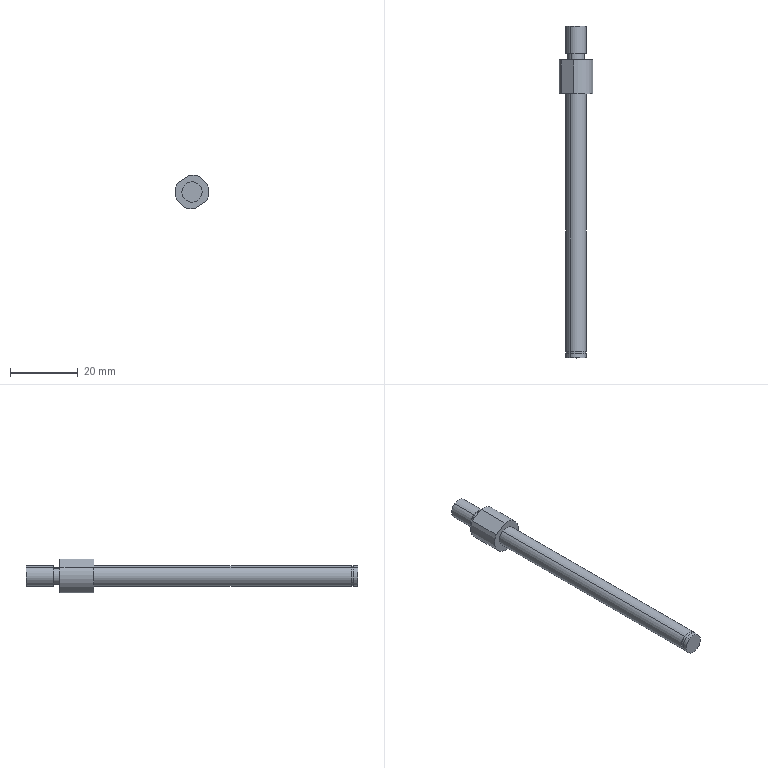Component | SolidWorks | JL001-03-06-1_JL001-03-06-001-1 | 1 solid | 21 faces | box 10 x 98 x 10 mm | volume 3225 mm3 | cylinder 12 | plane 9 | commonest cylinder face diameters 6 x6 5 x2 5.7 x2 10 x2
build123d program:
from build123d import *

# Parameters (mm, degrees)
SKETCH6_OUTSIDE_W   = 31.804
SKETCH6_OUTSIDE_H   = 31.804
SKETCH6_OUTSIDE_W_2 = 16.589
SKETCH6_OUTSIDE_H_2 = 9
CUT_EXTRUDE2_DEPTH  = 79.32


with BuildPart() as part:
    # Sketch1 → Revolve1 (revolve)
    with BuildSketch(Plane.XY, mode=Mode.PRIVATE) as revolve1_sk:
        Polygon((0, 98), (3, 98), (3, 96.8), (2.85, 96.8), (2.85, 96), (3, 96), (3, 20), (5, 20), (5, 10), (2.5, 10), (2.5, 8), (3, 8), (3, 0), (0, 0), align=None)
    revolve(revolve1_sk.sketch.rotate(Axis((0, 0, 0), (0, 1, 0)), 90), axis=Axis((0, 0, 0), (0, 1, 0)))

    # Sketch6 outside → Cut-Extrude2 (cut, through all)
    with BuildSketch(Plane(origin=(0, 20, 0), x_dir=(1, 0, 0), z_dir=(0, 1, 0))):
        Rectangle(SKETCH6_OUTSIDE_W, SKETCH6_OUTSIDE_H)
        Rectangle(SKETCH6_OUTSIDE_W_2, SKETCH6_OUTSIDE_H_2, mode=Mode.SUBTRACT)
    extrude(amount=-CUT_EXTRUDE2_DEPTH, mode=Mode.SUBTRACT)


solid = part.part

# Placed as in the assembly
solid = solid.moved(Location((-69, 1135, 65), (0, -33.158, 180)))
STEP:
#1=CARTESIAN_POINT('',(-2.781,44.37,2.658));
#2=VERTEX_POINT('',#1);
#3=CARTESIAN_POINT('',(-2.652,44.37,2.46));
#4=VERTEX_POINT('',#3);
#5=CARTESIAN_POINT('',(-2.717,44.37,2.559));
#6=DIRECTION('',(0.,1.,0.));
#7=DIRECTION('',(-0.5469,0.,0.8372));
#8=AXIS2_PLACEMENT_3D('',#5,#6,#7);
#9=CIRCLE('',#8,0.1181);
#10=EDGE_CURVE('',#2,#4,#9,.T.);
#11=ORIENTED_EDGE('',*,*,#10,.T.);
#12=CARTESIAN_POINT('',(-2.652,44.685,2.46));
#13=VERTEX_POINT('',#12);
#14=CARTESIAN_POINT('',(-2.652,44.685,2.46));
#15=DIRECTION('',(0.,1.,0.));
#16=VECTOR('',#15,39.37);
#17=LINE('',#14,#16);
#18=EDGE_CURVE('',#4,#13,#17,.T.);
#19=ORIENTED_EDGE('',*,*,#18,.T.);
#20=CARTESIAN_POINT('',(-2.781,44.685,2.658));
#21=VERTEX_POINT('',#20);
#22=CARTESIAN_POINT('',(-2.717,44.685,2.559));
#23=DIRECTION('',(0.,1.,0.));
#24=DIRECTION('',(-0.5469,0.,0.8372));
#25=AXIS2_PLACEMENT_3D('',#22,#23,#24);
#26=CIRCLE('',#25,0.1181);
#27=EDGE_CURVE('',#21,#13,#26,.T.);
#28=ORIENTED_EDGE('',*,*,#27,.F.);
#29=CARTESIAN_POINT('',(-2.781,44.685,2.658));
#30=DIRECTION('',(0.,1.,0.));
#31=VECTOR('',#30,39.37);
#32=LINE('',#29,#31);
#33=EDGE_CURVE('',#2,#21,#32,.T.);
#34=ORIENTED_EDGE('',*,*,#33,.F.);
#35=EDGE_LOOP('',(#11,#19,#28,#34));
#36=FACE_OUTER_BOUND('',#35,.T.);
#37=CARTESIAN_POINT('',(-2.717,44.685,2.559));
#38=DIRECTION('',(0.,1.,0.));
#39=DIRECTION('',(-0.5469,0.,0.8372));
#40=AXIS2_PLACEMENT_3D('',#37,#38,#39);
#41=CYLINDRICAL_SURFACE('',#40,0.1181);
#42=ADVANCED_FACE('',(#36),#41,.T.);
#43=CARTESIAN_POINT('',(-2.77,44.291,2.641));
#44=VERTEX_POINT('',#43);
#45=CARTESIAN_POINT('',(-2.663,44.291,2.477));
#46=VERTEX_POINT('',#45);
#47=CARTESIAN_POINT('',(-2.717,44.291,2.559));
#48=DIRECTION('',(0.,1.,0.));
#49=DIRECTION('',(-0.5469,0.,0.8372));
#50=AXIS2_PLACEMENT_3D('',#47,#48,#49);
#51=CIRCLE('',#50,0.09843);
#52=EDGE_CURVE('',#44,#46,#51,.T.);
#53=ORIENTED_EDGE('',*,*,#52,.T.);
#54=CARTESIAN_POINT('',(-2.663,44.37,2.477));
#55=VERTEX_POINT('',#54);
#56=CARTESIAN_POINT('',(-2.663,44.685,2.477));
#57=DIRECTION('',(0.,1.,0.));
#58=VECTOR('',#57,39.37);
#59=LINE('',#56,#58);
#60=EDGE_CURVE('',#46,#55,#59,.T.);
#61=ORIENTED_EDGE('',*,*,#60,.T.);
#62=CARTESIAN_POINT('',(-2.77,44.37,2.641));
#63=VERTEX_POINT('',#62);
#64=CARTESIAN_POINT('',(-2.717,44.37,2.559));
#65=DIRECTION('',(0.,1.,0.));
#66=DIRECTION('',(-0.5469,0.,0.8372));
#67=AXIS2_PLACEMENT_3D('',#64,#65,#66);
#68=CIRCLE('',#67,0.09843);
#69=EDGE_CURVE('',#63,#55,#68,.T.);
#70=ORIENTED_EDGE('',*,*,#69,.F.);
#71=CARTESIAN_POINT('',(-2.77,44.685,2.641));
#72=DIRECTION('',(0.,1.,0.));
#73=VECTOR('',#72,39.37);
#74=LINE('',#71,#73);
#75=EDGE_CURVE('',#44,#63,#74,.T.);
#76=ORIENTED_EDGE('',*,*,#75,.F.);
#77=EDGE_LOOP('',(#53,#61,#70,#76));
#78=FACE_OUTER_BOUND('',#77,.T.);
#79=CARTESIAN_POINT('',(-2.717,44.685,2.559));
#80=DIRECTION('',(0.,1.,0.));
#81=DIRECTION('',(-0.5469,0.,0.8372));
#82=AXIS2_PLACEMENT_3D('',#79,#80,#81);
#83=CYLINDRICAL_SURFACE('',#82,0.09843);
#84=ADVANCED_FACE('',(#78),#83,.T.);
#85=CARTESIAN_POINT('',(-2.781,40.906,2.658));
#86=VERTEX_POINT('',#85);
#87=CARTESIAN_POINT('',(-2.652,40.906,2.46));
#88=VERTEX_POINT('',#87);
#89=CARTESIAN_POINT('',(-2.717,40.906,2.559));
#90=DIRECTION('',(0.,1.,0.));
#91=DIRECTION('',(-0.5469,0.,0.8372));
#92=AXIS2_PLACEMENT_3D('',#89,#90,#91);
#93=CIRCLE('',#92,0.1181);
#94=EDGE_CURVE('',#86,#88,#93,.T.);
#95=ORIENTED_EDGE('',*,*,#94,.T.);
#96=CARTESIAN_POINT('',(-2.652,43.898,2.46));
#97=VERTEX_POINT('',#96);
#98=CARTESIAN_POINT('',(-2.652,44.685,2.46));
#99=DIRECTION('',(0.,1.,0.));
#100=VECTOR('',#99,39.37);
#101=LINE('',#98,#100);
#102=EDGE_CURVE('',#88,#97,#101,.T.);
#103=ORIENTED_EDGE('',*,*,#102,.T.);
#104=CARTESIAN_POINT('',(-2.781,43.898,2.658));
#105=VERTEX_POINT('',#104);
#106=CARTESIAN_POINT('',(-2.717,43.898,2.559));
#107=DIRECTION('',(0.,1.,0.));
#108=DIRECTION('',(-0.5469,0.,0.8372));
#109=AXIS2_PLACEMENT_3D('',#106,#107,#108);
#110=CIRCLE('',#109,0.1181);
#111=EDGE_CURVE('',#105,#97,#110,.T.);
#112=ORIENTED_EDGE('',*,*,#111,.F.);
#113=CARTESIAN_POINT('',(-2.781,44.685,2.658));
#114=DIRECTION('',(0.,1.,0.));
#115=VECTOR('',#114,39.37);
#116=LINE('',#113,#115);
#117=EDGE_CURVE('',#86,#105,#116,.T.);
#118=ORIENTED_EDGE('',*,*,#117,.F.);
#119=EDGE_LOOP('',(#95,#103,#112,#118));
#120=FACE_OUTER_BOUND('',#119,.T.);
#121=CARTESIAN_POINT('',(-2.717,44.685,2.559));
#122=DIRECTION('',(0.,1.,0.));
#123=DIRECTION('',(-0.5469,0.,0.8372));
#124=AXIS2_PLACEMENT_3D('',#121,#122,#123);
#125=CYLINDRICAL_SURFACE('',#124,0.1181);
#126=ADVANCED_FACE('',(#120),#125,.T.);
#127=CARTESIAN_POINT('',(-2.778,40.874,2.653));
#128=VERTEX_POINT('',#127);
#129=CARTESIAN_POINT('',(-2.655,40.874,2.465));
#130=VERTEX_POINT('',#129);
#131=CARTESIAN_POINT('',(-2.717,40.874,2.559));
#132=DIRECTION('',(0.,1.,0.));
#133=DIRECTION('',(-0.5469,0.,0.8372));
#134=AXIS2_PLACEMENT_3D('',#131,#132,#133);
#135=CIRCLE('',#134,0.1122);
#136=EDGE_CURVE('',#128,#130,#135,.T.);
#137=ORIENTED_EDGE('',*,*,#136,.T.);
#138=CARTESIAN_POINT('',(-2.655,40.906,2.465));
#139=VERTEX_POINT('',#138);
#140=CARTESIAN_POINT('',(-2.655,44.685,2.465));
#141=DIRECTION('',(0.,1.,0.));
#142=VECTOR('',#141,39.37);
#143=LINE('',#140,#142);
#144=EDGE_CURVE('',#130,#139,#143,.T.);
#145=ORIENTED_EDGE('',*,*,#144,.T.);
#146=CARTESIAN_POINT('',(-2.778,40.906,2.653));
#147=VERTEX_POINT('',#146);
#148=CARTESIAN_POINT('',(-2.717,40.906,2.559));
#149=DIRECTION('',(0.,1.,0.));
#150=DIRECTION('',(-0.5469,0.,0.8372));
#151=AXIS2_PLACEMENT_3D('',#148,#149,#150);
#152=CIRCLE('',#151,0.1122);
#153=EDGE_CURVE('',#147,#139,#152,.T.);
#154=ORIENTED_EDGE('',*,*,#153,.F.);
#155=CARTESIAN_POINT('',(-2.778,44.685,2.653));
#156=DIRECTION('',(0.,1.,0.));
#157=VECTOR('',#156,39.37);
#158=LINE('',#155,#157);
#159=EDGE_CURVE('',#128,#147,#158,.T.);
#160=ORIENTED_EDGE('',*,*,#159,.F.);
#161=EDGE_LOOP('',(#137,#145,#154,#160));
#162=FACE_OUTER_BOUND('',#161,.T.);
#163=CARTESIAN_POINT('',(-2.717,44.685,2.559));
#164=DIRECTION('',(0.,1.,0.));
#165=DIRECTION('',(-0.5469,0.,0.8372));
#166=AXIS2_PLACEMENT_3D('',#163,#164,#165);
#167=CYLINDRICAL_SURFACE('',#166,0.1122);
#168=ADVANCED_FACE('',(#162),#167,.T.);
#169=CARTESIAN_POINT('',(-2.781,40.827,2.658));
#170=VERTEX_POINT('',#169);
#171=CARTESIAN_POINT('',(-2.652,40.827,2.46));
#172=VERTEX_POINT('',#171);
#173=CARTESIAN_POINT('',(-2.717,40.827,2.559));
#174=DIRECTION('',(0.,1.,0.));
#175=DIRECTION('',(-0.5469,0.,0.8372));
#176=AXIS2_PLACEMENT_3D('',#173,#174,#175);
#177=CIRCLE('',#176,0.1181);
#178=EDGE_CURVE('',#170,#172,#177,.T.);
#179=ORIENTED_EDGE('',*,*,#178,.T.);
#180=CARTESIAN_POINT('',(-2.652,40.874,2.46));
#181=VERTEX_POINT('',#180);
#182=CARTESIAN_POINT('',(-2.652,44.685,2.46));
#183=DIRECTION('',(0.,1.,0.));
#184=VECTOR('',#183,39.37);
#185=LINE('',#182,#184);
#186=EDGE_CURVE('',#172,#181,#185,.T.);
#187=ORIENTED_EDGE('',*,*,#186,.T.);
#188=CARTESIAN_POINT('',(-2.781,40.874,2.658));
#189=VERTEX_POINT('',#188);
#190=CARTESIAN_POINT('',(-2.717,40.874,2.559));
#191=DIRECTION('',(0.,1.,0.));
#192=DIRECTION('',(-0.5469,0.,0.8372));
#193=AXIS2_PLACEMENT_3D('',#190,#191,#192);
#194=CIRCLE('',#193,0.1181);
#195=EDGE_CURVE('',#189,#181,#194,.T.);
#196=ORIENTED_EDGE('',*,*,#195,.F.);
#197=CARTESIAN_POINT('',(-2.781,44.685,2.658));
#198=DIRECTION('',(0.,1.,0.));
#199=VECTOR('',#198,39.37);
#200=LINE('',#197,#199);
#201=EDGE_CURVE('',#170,#189,#200,.T.);
#202=ORIENTED_EDGE('',*,*,#201,.F.);
#203=EDGE_LOOP('',(#179,#187,#196,#202));
#204=FACE_OUTER_BOUND('',#203,.T.);
#205=CARTESIAN_POINT('',(-2.717,44.685,2.559));
#206=DIRECTION('',(0.,1.,0.));
#207=DIRECTION('',(-0.5469,0.,0.8372));
#208=AXIS2_PLACEMENT_3D('',#205,#206,#207);
#209=CYLINDRICAL_SURFACE('',#208,0.1181);
#210=ADVANCED_FACE('',(#204),#209,.T.);
#211=ORIENTED_EDGE('',*,*,#111,.T.);
#212=CARTESIAN_POINT('',(-2.717,43.898,2.559));
#213=DIRECTION('',(0.,1.,0.));
#214=DIRECTION('',(-0.5469,0.,0.8372));
#215=AXIS2_PLACEMENT_3D('',#212,#213,#214);
#216=CIRCLE('',#215,0.1181);
#217=EDGE_CURVE('',#97,#105,#216,.T.);
#218=ORIENTED_EDGE('',*,*,#217,.T.);
#219=EDGE_LOOP('',(#211,#218));
#220=FACE_BOUND('',#219,.T.);
#221=CARTESIAN_POINT('',(-2.691,43.898,2.364));
#222=VERTEX_POINT('',#221);
#223=CARTESIAN_POINT('',(-2.885,43.898,2.66));
#224=VERTEX_POINT('',#223);
#225=CARTESIAN_POINT('',(-2.717,43.898,2.559));
#226=DIRECTION('',(0.,1.,0.));
#227=DIRECTION('',(-0.5469,0.,0.8372));
#228=AXIS2_PLACEMENT_3D('',#225,#226,#227);
#229=CIRCLE('',#228,0.1969);
#230=EDGE_CURVE('',#222,#224,#229,.T.);
#231=ORIENTED_EDGE('',*,*,#230,.F.);
#232=CARTESIAN_POINT('',(-2.548,43.898,2.458));
#233=VERTEX_POINT('',#232);
#234=CARTESIAN_POINT('',(-2.893,43.898,2.232));
#235=DIRECTION('',(0.8372,-0.,0.5469));
#236=VECTOR('',#235,39.37);
#237=LINE('',#234,#236);
#238=EDGE_CURVE('',#222,#233,#237,.T.);
#239=ORIENTED_EDGE('',*,*,#238,.T.);
#240=CARTESIAN_POINT('',(-2.742,43.898,2.754));
#241=VERTEX_POINT('',#240);
#242=CARTESIAN_POINT('',(-2.717,43.898,2.559));
#243=DIRECTION('',(0.,1.,0.));
#244=DIRECTION('',(-0.5469,0.,0.8372));
#245=AXIS2_PLACEMENT_3D('',#242,#243,#244);
#246=CIRCLE('',#245,0.1969);
#247=EDGE_CURVE('',#241,#233,#246,.T.);
#248=ORIENTED_EDGE('',*,*,#247,.F.);
#249=CARTESIAN_POINT('',(-3.087,43.898,2.529));
#250=DIRECTION('',(-0.8372,0.,-0.5469));
#251=VECTOR('',#250,39.37);
#252=LINE('',#249,#251);
#253=EDGE_CURVE('',#241,#224,#252,.T.);
#254=ORIENTED_EDGE('',*,*,#253,.T.);
#255=EDGE_LOOP('',(#231,#239,#248,#254));
#256=FACE_OUTER_BOUND('',#255,.T.);
#257=CARTESIAN_POINT('',(-2.618,43.898,2.624));
#258=DIRECTION('',(0.,-1.,-0.));
#259=DIRECTION('',(0.5469,0.,-0.8372));
#260=AXIS2_PLACEMENT_3D('',#257,#258,#259);
#261=PLANE('',#260);
#262=ADVANCED_FACE('',(#220,#256),#261,.T.);
#263=CARTESIAN_POINT('',(-2.691,44.291,2.364));
#264=VERTEX_POINT('',#263);
#265=CARTESIAN_POINT('',(-2.885,44.291,2.66));
#266=VERTEX_POINT('',#265);
#267=CARTESIAN_POINT('',(-2.717,44.291,2.559));
#268=DIRECTION('',(0.,1.,0.));
#269=DIRECTION('',(-0.5469,0.,0.8372));
#270=AXIS2_PLACEMENT_3D('',#267,#268,#269);
#271=CIRCLE('',#270,0.1969);
#272=EDGE_CURVE('',#264,#266,#271,.T.);
#273=ORIENTED_EDGE('',*,*,#272,.F.);
#274=CARTESIAN_POINT('',(-2.691,44.685,2.364));
#275=DIRECTION('',(-0.,-1.,-0.));
#276=VECTOR('',#275,39.37);
#277=LINE('',#274,#276);
#278=EDGE_CURVE('',#264,#222,#277,.T.);
#279=ORIENTED_EDGE('',*,*,#278,.T.);
#280=ORIENTED_EDGE('',*,*,#230,.T.);
#281=CARTESIAN_POINT('',(-2.885,44.685,2.66));
#282=DIRECTION('',(0.,1.,0.));
#283=VECTOR('',#282,39.37);
#284=LINE('',#281,#283);
#285=EDGE_CURVE('',#224,#266,#284,.T.);
#286=ORIENTED_EDGE('',*,*,#285,.T.);
#287=EDGE_LOOP('',(#273,#279,#280,#286));
#288=FACE_OUTER_BOUND('',#287,.T.);
#289=CARTESIAN_POINT('',(-2.717,44.685,2.559));
#290=DIRECTION('',(0.,1.,0.));
#291=DIRECTION('',(-0.5469,0.,0.8372));
#292=AXIS2_PLACEMENT_3D('',#289,#290,#291);
#293=CYLINDRICAL_SURFACE('',#292,0.1969);
#294=ADVANCED_FACE('',(#288),#293,.T.);
#295=ORIENTED_EDGE('',*,*,#247,.T.);
#296=CARTESIAN_POINT('',(-2.548,44.291,2.458));
#297=VERTEX_POINT('',#296);
#298=CARTESIAN_POINT('',(-2.548,44.685,2.458));
#299=DIRECTION('',(0.,1.,0.));
#300=VECTOR('',#299,39.37);
#301=LINE('',#298,#300);
#302=EDGE_CURVE('',#233,#297,#301,.T.);
#303=ORIENTED_EDGE('',*,*,#302,.T.);
#304=CARTESIAN_POINT('',(-2.742,44.291,2.754));
#305=VERTEX_POINT('',#304);
#306=CARTESIAN_POINT('',(-2.717,44.291,2.559));
#307=DIRECTION('',(0.,1.,0.));
#308=DIRECTION('',(-0.5469,0.,0.8372));
#309=AXIS2_PLACEMENT_3D('',#306,#307,#308);
#310=CIRCLE('',#309,0.1969);
#311=EDGE_CURVE('',#305,#297,#310,.T.);
#312=ORIENTED_EDGE('',*,*,#311,.F.);
#313=CARTESIAN_POINT('',(-2.742,44.685,2.754));
#314=DIRECTION('',(-0.,-1.,-0.));
#315=VECTOR('',#314,39.37);
#316=LINE('',#313,#315);
#317=EDGE_CURVE('',#305,#241,#316,.T.);
#318=ORIENTED_EDGE('',*,*,#317,.T.);
#319=EDGE_LOOP('',(#295,#303,#312,#318));
#320=FACE_OUTER_BOUND('',#319,.T.);
#321=CARTESIAN_POINT('',(-2.717,44.685,2.559));
#322=DIRECTION('',(0.,1.,0.));
#323=DIRECTION('',(-0.5469,0.,0.8372));
#324=AXIS2_PLACEMENT_3D('',#321,#322,#323);
#325=CYLINDRICAL_SURFACE('',#324,0.1969);
#326=ADVANCED_FACE('',(#320),#325,.T.);
#327=ORIENTED_EDGE('',*,*,#52,.F.);
#328=CARTESIAN_POINT('',(-2.717,44.291,2.559));
#329=DIRECTION('',(0.,1.,0.));
#330=DIRECTION('',(-0.5469,0.,0.8372));
#331=AXIS2_PLACEMENT_3D('',#328,#329,#330);
#332=CIRCLE('',#331,0.09843);
#333=EDGE_CURVE('',#46,#44,#332,.T.);
#334=ORIENTED_EDGE('',*,*,#333,.F.);
#335=EDGE_LOOP('',(#327,#334));
#336=FACE_BOUND('',#335,.T.);
#337=ORIENTED_EDGE('',*,*,#311,.T.);
#338=CARTESIAN_POINT('',(-2.455,44.291,2.518));
#339=DIRECTION('',(-0.8372,0.,-0.5469));
#340=VECTOR('',#339,39.37);
#341=LINE('',#338,#340);
#342=EDGE_CURVE('',#297,#264,#341,.T.);
#343=ORIENTED_EDGE('',*,*,#342,.T.);
#344=ORIENTED_EDGE('',*,*,#272,.T.);
#345=CARTESIAN_POINT('',(-2.649,44.291,2.815));
#346=DIRECTION('',(0.8372,-0.,0.5469));
#347=VECTOR('',#346,39.37);
#348=LINE('',#345,#347);
#349=EDGE_CURVE('',#266,#305,#348,.T.);
#350=ORIENTED_EDGE('',*,*,#349,.T.);
#351=EDGE_LOOP('',(#337,#343,#344,#350));
#352=FACE_OUTER_BOUND('',#351,.T.);
#353=CARTESIAN_POINT('',(-2.552,44.291,2.667));
#354=DIRECTION('',(-0.,1.,0.));
#355=DIRECTION('',(-0.5469,-0.,0.8372));
#356=AXIS2_PLACEMENT_3D('',#353,#354,#355);
#357=PLANE('',#356);
#358=ADVANCED_FACE('',(#336,#352),#357,.T.);
#359=ORIENTED_EDGE('',*,*,#178,.F.);
#360=CARTESIAN_POINT('',(-2.717,40.827,2.559));
#361=DIRECTION('',(0.,1.,0.));
#362=DIRECTION('',(-0.5469,0.,0.8372));
#363=AXIS2_PLACEMENT_3D('',#360,#361,#362);
#364=CIRCLE('',#363,0.1181);
#365=EDGE_CURVE('',#172,#170,#364,.T.);
#366=ORIENTED_EDGE('',*,*,#365,.F.);
#367=EDGE_LOOP('',(#359,#366));
#368=FACE_OUTER_BOUND('',#367,.T.);
#369=CARTESIAN_POINT('',(-2.717,40.827,2.559));
#370=DIRECTION('',(0.,-1.,-0.));
#371=DIRECTION('',(0.5469,0.,-0.8372));
#372=AXIS2_PLACEMENT_3D('',#369,#370,#371);
#373=PLANE('',#372);
#374=ADVANCED_FACE('',(#368),#373,.T.);
#375=ORIENTED_EDGE('',*,*,#186,.F.);
#376=ORIENTED_EDGE('',*,*,#365,.T.);
#377=ORIENTED_EDGE('',*,*,#201,.T.);
#378=CARTESIAN_POINT('',(-2.717,40.874,2.559));
#379=DIRECTION('',(0.,1.,0.));
#380=DIRECTION('',(-0.5469,0.,0.8372));
#381=AXIS2_PLACEMENT_3D('',#378,#379,#380);
#382=CIRCLE('',#381,0.1181);
#383=EDGE_CURVE('',#181,#189,#382,.T.);
#384=ORIENTED_EDGE('',*,*,#383,.F.);
#385=EDGE_LOOP('',(#375,#376,#377,#384));
#386=FACE_OUTER_BOUND('',#385,.T.);
#387=CARTESIAN_POINT('',(-2.717,44.685,2.559));
#388=DIRECTION('',(0.,1.,0.));
#389=DIRECTION('',(-0.5469,0.,0.8372));
#390=AXIS2_PLACEMENT_3D('',#387,#388,#389);
#391=CYLINDRICAL_SURFACE('',#390,0.1181);
#392=ADVANCED_FACE('',(#386),#391,.T.);
#393=ORIENTED_EDGE('',*,*,#195,.T.);
#394=ORIENTED_EDGE('',*,*,#383,.T.);
#395=EDGE_LOOP('',(#393,#394));
#396=FACE_OUTER_BOUND('',#395,.T.);
#397=ORIENTED_EDGE('',*,*,#136,.F.);
#398=CARTESIAN_POINT('',(-2.717,40.874,2.559));
#399=DIRECTION('',(0.,1.,0.));
#400=DIRECTION('',(-0.5469,0.,0.8372));
#401=AXIS2_PLACEMENT_3D('',#398,#399,#400);
#402=CIRCLE('',#401,0.1122);
#403=EDGE_CURVE('',#130,#128,#402,.T.);
#404=ORIENTED_EDGE('',*,*,#403,.F.);
#405=EDGE_LOOP('',(#397,#404));
#406=FACE_BOUND('',#405,.T.);
#407=CARTESIAN_POINT('',(-2.618,40.874,2.624));
#408=DIRECTION('',(-0.,1.,0.));
#409=DIRECTION('',(-0.5469,-0.,0.8372));
#410=AXIS2_PLACEMENT_3D('',#407,#408,#409);
#411=PLANE('',#410);
#412=ADVANCED_FACE('',(#396,#406),#411,.T.);
#413=ORIENTED_EDGE('',*,*,#144,.F.);
#414=ORIENTED_EDGE('',*,*,#403,.T.);
#415=ORIENTED_EDGE('',*,*,#159,.T.);
#416=CARTESIAN_POINT('',(-2.717,40.906,2.559));
#417=DIRECTION('',(0.,1.,0.));
#418=DIRECTION('',(-0.5469,0.,0.8372));
#419=AXIS2_PLACEMENT_3D('',#416,#417,#418);
#420=CIRCLE('',#419,0.1122);
#421=EDGE_CURVE('',#139,#147,#420,.T.);
#422=ORIENTED_EDGE('',*,*,#421,.F.);
#423=EDGE_LOOP('',(#413,#414,#415,#422));
#424=FACE_OUTER_BOUND('',#423,.T.);
#425=CARTESIAN_POINT('',(-2.717,44.685,2.559));
#426=DIRECTION('',(0.,1.,0.));
#427=DIRECTION('',(-0.5469,0.,0.8372));
#428=AXIS2_PLACEMENT_3D('',#425,#426,#427);
#429=CYLINDRICAL_SURFACE('',#428,0.1122);
#430=ADVANCED_FACE('',(#424),#429,.T.);
#431=ORIENTED_EDGE('',*,*,#153,.T.);
#432=ORIENTED_EDGE('',*,*,#421,.T.);
#433=EDGE_LOOP('',(#431,#432));
#434=FACE_BOUND('',#433,.T.);
#435=ORIENTED_EDGE('',*,*,#94,.F.);
#436=CARTESIAN_POINT('',(-2.717,40.906,2.559));
#437=DIRECTION('',(0.,1.,0.));
#438=DIRECTION('',(-0.5469,0.,0.8372));
#439=AXIS2_PLACEMENT_3D('',#436,#437,#438);
#440=CIRCLE('',#439,0.1181);
#441=EDGE_CURVE('',#88,#86,#440,.T.);
#442=ORIENTED_EDGE('',*,*,#441,.F.);
#443=EDGE_LOOP('',(#435,#442));
#444=FACE_OUTER_BOUND('',#443,.T.);
#445=CARTESIAN_POINT('',(-2.623,40.906,2.62));
#446=DIRECTION('',(0.,-1.,-0.));
#447=DIRECTION('',(0.5469,0.,-0.8372));
#448=AXIS2_PLACEMENT_3D('',#445,#446,#447);
#449=PLANE('',#448);
#450=ADVANCED_FACE('',(#434,#444),#449,.T.);
#451=ORIENTED_EDGE('',*,*,#102,.F.);
#452=ORIENTED_EDGE('',*,*,#441,.T.);
#453=ORIENTED_EDGE('',*,*,#117,.T.);
#454=ORIENTED_EDGE('',*,*,#217,.F.);
#455=EDGE_LOOP('',(#451,#452,#453,#454));
#456=FACE_OUTER_BOUND('',#455,.T.);
#457=CARTESIAN_POINT('',(-2.717,44.685,2.559));
#458=DIRECTION('',(0.,1.,0.));
#459=DIRECTION('',(-0.5469,0.,0.8372));
#460=AXIS2_PLACEMENT_3D('',#457,#458,#459);
#461=CYLINDRICAL_SURFACE('',#460,0.1181);
#462=ADVANCED_FACE('',(#456),#461,.T.);
#463=ORIENTED_EDGE('',*,*,#60,.F.);
#464=ORIENTED_EDGE('',*,*,#333,.T.);
#465=ORIENTED_EDGE('',*,*,#75,.T.);
#466=CARTESIAN_POINT('',(-2.717,44.37,2.559));
#467=DIRECTION('',(0.,1.,0.));
#468=DIRECTION('',(-0.5469,0.,0.8372));
#469=AXIS2_PLACEMENT_3D('',#466,#467,#468);
#470=CIRCLE('',#469,0.09843);
#471=EDGE_CURVE('',#55,#63,#470,.T.);
#472=ORIENTED_EDGE('',*,*,#471,.F.);
#473=EDGE_LOOP('',(#463,#464,#465,#472));
#474=FACE_OUTER_BOUND('',#473,.T.);
#475=CARTESIAN_POINT('',(-2.717,44.685,2.559));
#476=DIRECTION('',(0.,1.,0.));
#477=DIRECTION('',(-0.5469,0.,0.8372));
#478=AXIS2_PLACEMENT_3D('',#475,#476,#477);
#479=CYLINDRICAL_SURFACE('',#478,0.09843);
#480=ADVANCED_FACE('',(#474),#479,.T.);
#481=ORIENTED_EDGE('',*,*,#69,.T.);
#482=ORIENTED_EDGE('',*,*,#471,.T.);
#483=EDGE_LOOP('',(#481,#482));
#484=FACE_BOUND('',#483,.T.);
#485=ORIENTED_EDGE('',*,*,#10,.F.);
#486=CARTESIAN_POINT('',(-2.717,44.37,2.559));
#487=DIRECTION('',(0.,1.,0.));
#488=DIRECTION('',(-0.5469,0.,0.8372));
#489=AXIS2_PLACEMENT_3D('',#486,#487,#488);
#490=CIRCLE('',#489,0.1181);
#491=EDGE_CURVE('',#4,#2,#490,.T.);
#492=ORIENTED_EDGE('',*,*,#491,.F.);
#493=EDGE_LOOP('',(#485,#492));
#494=FACE_OUTER_BOUND('',#493,.T.);
#495=CARTESIAN_POINT('',(-2.634,44.37,2.613));
#496=DIRECTION('',(0.,-1.,-0.));
#497=DIRECTION('',(0.5469,0.,-0.8372));
#498=AXIS2_PLACEMENT_3D('',#495,#496,#497);
#499=PLANE('',#498);
#500=ADVANCED_FACE('',(#484,#494),#499,.T.);
#501=ORIENTED_EDGE('',*,*,#18,.F.);
#502=ORIENTED_EDGE('',*,*,#491,.T.);
#503=ORIENTED_EDGE('',*,*,#33,.T.);
#504=CARTESIAN_POINT('',(-2.717,44.685,2.559));
#505=DIRECTION('',(0.,1.,0.));
#506=DIRECTION('',(-0.5469,0.,0.8372));
#507=AXIS2_PLACEMENT_3D('',#504,#505,#506);
#508=CIRCLE('',#507,0.1181);
#509=EDGE_CURVE('',#13,#21,#508,.T.);
#510=ORIENTED_EDGE('',*,*,#509,.F.);
#511=EDGE_LOOP('',(#501,#502,#503,#510));
#512=FACE_OUTER_BOUND('',#511,.T.);
#513=CARTESIAN_POINT('',(-2.717,44.685,2.559));
#514=DIRECTION('',(0.,1.,0.));
#515=DIRECTION('',(-0.5469,0.,0.8372));
#516=AXIS2_PLACEMENT_3D('',#513,#514,#515);
#517=CYLINDRICAL_SURFACE('',#516,0.1181);
#518=ADVANCED_FACE('',(#512),#517,.T.);
#519=ORIENTED_EDGE('',*,*,#27,.T.);
#520=ORIENTED_EDGE('',*,*,#509,.T.);
#521=EDGE_LOOP('',(#519,#520));
#522=FACE_OUTER_BOUND('',#521,.T.);
#523=CARTESIAN_POINT('',(-2.618,44.685,2.624));
#524=DIRECTION('',(-0.,1.,0.));
#525=DIRECTION('',(-0.5469,-0.,0.8372));
#526=AXIS2_PLACEMENT_3D('',#523,#524,#525);
#527=PLANE('',#526);
#528=ADVANCED_FACE('',(#522),#527,.T.);
#529=ORIENTED_EDGE('',*,*,#349,.F.);
#530=ORIENTED_EDGE('',*,*,#285,.F.);
#531=ORIENTED_EDGE('',*,*,#253,.F.);
#532=ORIENTED_EDGE('',*,*,#317,.F.);
#533=EDGE_LOOP('',(#529,#530,#531,#532));
#534=FACE_OUTER_BOUND('',#533,.T.);
#535=CARTESIAN_POINT('',(-3.087,44.685,2.529));
#536=DIRECTION('',(-0.5469,-0.,0.8372));
#537=DIRECTION('',(-0.8372,0.,-0.5469));
#538=AXIS2_PLACEMENT_3D('',#535,#536,#537);
#539=PLANE('',#538);
#540=ADVANCED_FACE('',(#534),#539,.T.);
#541=ORIENTED_EDGE('',*,*,#342,.F.);
#542=ORIENTED_EDGE('',*,*,#302,.F.);
#543=ORIENTED_EDGE('',*,*,#238,.F.);
#544=ORIENTED_EDGE('',*,*,#278,.F.);
#545=EDGE_LOOP('',(#541,#542,#543,#544));
#546=FACE_OUTER_BOUND('',#545,.T.);
#547=CARTESIAN_POINT('',(-2.893,44.685,2.232));
#548=DIRECTION('',(0.5469,0.,-0.8372));
#549=DIRECTION('',(0.8372,-0.,0.5469));
#550=AXIS2_PLACEMENT_3D('',#547,#548,#549);
#551=PLANE('',#550);
#552=ADVANCED_FACE('',(#546),#551,.T.);
#553=CLOSED_SHELL('',(#42,#84,#126,#168,#210,#262,#294,#326,#358,#374,#392,#412,#430,#450,#462,#480,#500,#518,#528,#540,#552));
#554=MANIFOLD_SOLID_BREP('',#553);
#555=CARTESIAN_POINT('',(0.,0.,0.));
#556=DIRECTION('',(0.,0.,1.));
#557=DIRECTION('',(1.,0.,0.));
#558=AXIS2_PLACEMENT_3D('',#555,#556,#557);
#559=(LENGTH_UNIT()NAMED_UNIT(*)SI_UNIT($,.METRE.));
#560=LENGTH_MEASURE_WITH_UNIT(LENGTH_MEASURE(0.0254),#559);
#561=DIMENSIONAL_EXPONENTS(1.,0.,0.,0.,0.,0.,0.);
#562=(CONVERSION_BASED_UNIT('',#560)LENGTH_UNIT()NAMED_UNIT(#561));
#563=UNCERTAINTY_MEASURE_WITH_UNIT(LENGTH_MEASURE(0.00001),#562,'','');
#564=(NAMED_UNIT(*)PLANE_ANGLE_UNIT()SI_UNIT($,.RADIAN.));
#565=(NAMED_UNIT(*)SI_UNIT($,.STERADIAN.)SOLID_ANGLE_UNIT());
#566=(GEOMETRIC_REPRESENTATION_CONTEXT(3)GLOBAL_UNCERTAINTY_ASSIGNED_CONTEXT((#563))GLOBAL_UNIT_ASSIGNED_CONTEXT((#562,#564,#565))REPRESENTATION_CONTEXT('',''));
#567=ADVANCED_BREP_SHAPE_REPRESENTATION('',(#554,#558),#566);
#568=COLOUR_RGB('',0.7922,0.8196,0.9333);
#569=FILL_AREA_STYLE_COLOUR('',#568);
#570=FILL_AREA_STYLE('',(#569));
#571=SURFACE_STYLE_FILL_AREA(#570);
#572=SURFACE_SIDE_STYLE('',(#571));
#573=SURFACE_STYLE_USAGE(.BOTH.,#572);
#574=PRESENTATION_STYLE_ASSIGNMENT((#573));
#575=STYLED_ITEM('',(#574),#554);
#576=PRESENTATION_LAYER_ASSIGNMENT('','',(#575));
#577=(LENGTH_UNIT()NAMED_UNIT(*)SI_UNIT($,.METRE.));
#578=LENGTH_MEASURE_WITH_UNIT(LENGTH_MEASURE(0.0254),#577);
#579=DIMENSIONAL_EXPONENTS(1.,0.,0.,0.,0.,0.,0.);
#580=(CONVERSION_BASED_UNIT('',#578)LENGTH_UNIT()NAMED_UNIT(#579));
#581=UNCERTAINTY_MEASURE_WITH_UNIT(LENGTH_MEASURE(0.00001),#580,'','');
#582=(NAMED_UNIT(*)PLANE_ANGLE_UNIT()SI_UNIT($,.RADIAN.));
#583=(NAMED_UNIT(*)SI_UNIT($,.STERADIAN.)SOLID_ANGLE_UNIT());
#584=(GEOMETRIC_REPRESENTATION_CONTEXT(3)GLOBAL_UNCERTAINTY_ASSIGNED_CONTEXT((#581))GLOBAL_UNIT_ASSIGNED_CONTEXT((#580,#582,#583))REPRESENTATION_CONTEXT('',''));
#585=MECHANICAL_DESIGN_GEOMETRIC_PRESENTATION_REPRESENTATION('',(#575),#584);